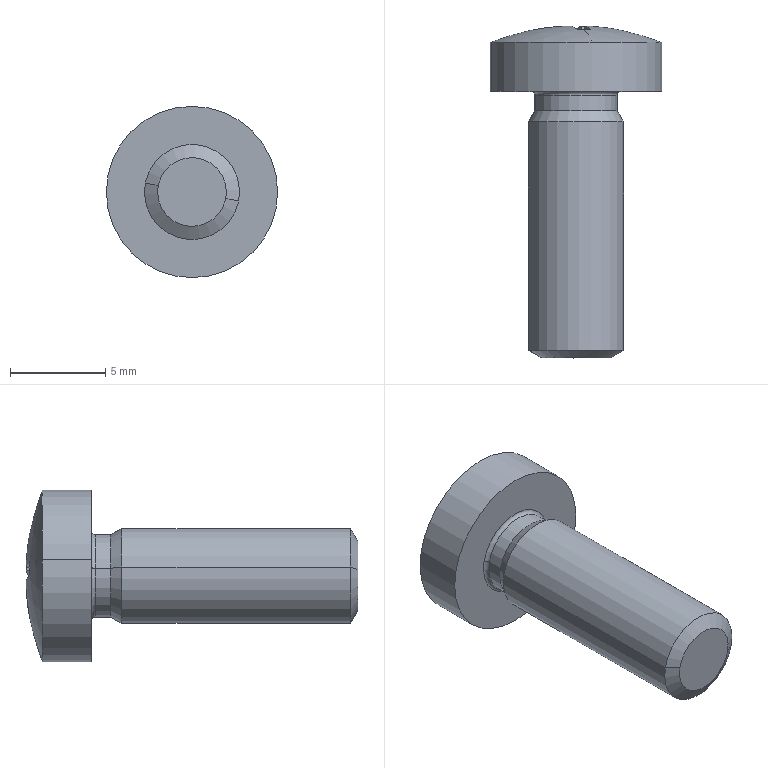Component | SolidWorks | GB823-88PhillipsSmallPanHeadScrewM5_14-1 | 1 solid | 28 faces | box 9 x 17.44 x 9 mm | volume 453 mm3 | plane 14 | cylinder 6 | cone 4 | torus 2 | sphere 2 | commonest cylinder face diameters 4.33 x2 9 x2 5 x2
STEP:
#1=COLOUR_RGB('',0.7922,0.8196,0.9333);
#2=FILL_AREA_STYLE_COLOUR('',#1);
#3=FILL_AREA_STYLE('',(#2));
#4=SURFACE_STYLE_FILL_AREA(#3);
#5=SURFACE_SIDE_STYLE('',(#4));
#6=SURFACE_STYLE_USAGE(.BOTH.,#5);
#7=PRESENTATION_STYLE_ASSIGNMENT((#6));
#8=CARTESIAN_POINT('',(-4.855,2.688,-4.337));
#9=VERTEX_POINT('',#8);
#10=CARTESIAN_POINT('',(-4.715,2.688,-4.364));
#11=VERTEX_POINT('',#10);
#12=CARTESIAN_POINT('',(-4.785,2.688,-4.351));
#13=DIRECTION('',(0.,1.,0.));
#14=DIRECTION('',(-0.9822,0.,0.188));
#15=AXIS2_PLACEMENT_3D('',#12,#13,#14);
#16=CIRCLE('',#15,0.07115);
#17=EDGE_CURVE('',#9,#11,#16,.T.);
#18=ORIENTED_EDGE('',*,*,#17,.T.);
#19=CARTESIAN_POINT('',(-4.688,2.704,-4.369));
#20=VERTEX_POINT('',#19);
#21=CARTESIAN_POINT('',(-4.688,2.704,-4.369));
#22=DIRECTION('',(0.8483,0.5041,-0.1623));
#23=VECTOR('',#22,39.37);
#24=LINE('',#21,#23);
#25=EDGE_CURVE('',#11,#20,#24,.T.);
#26=ORIENTED_EDGE('',*,*,#25,.T.);
#27=CARTESIAN_POINT('',(-4.881,2.704,-4.332));
#28=VERTEX_POINT('',#27);
#29=CARTESIAN_POINT('',(-4.785,2.704,-4.351));
#30=DIRECTION('',(0.,1.,0.));
#31=DIRECTION('',(-0.9822,0.,0.188));
#32=AXIS2_PLACEMENT_3D('',#29,#30,#31);
#33=CIRCLE('',#32,0.09843);
#34=EDGE_CURVE('',#28,#20,#33,.T.);
#35=ORIENTED_EDGE('',*,*,#34,.F.);
#36=CARTESIAN_POINT('',(-4.881,2.704,-4.332));
#37=DIRECTION('',(-0.8483,0.5041,0.1623));
#38=VECTOR('',#37,39.37);
#39=LINE('',#36,#38);
#40=EDGE_CURVE('',#9,#28,#39,.T.);
#41=ORIENTED_EDGE('',*,*,#40,.F.);
#42=EDGE_LOOP('',(#18,#26,#35,#41));
#43=FACE_OUTER_BOUND('',#42,.T.);
#44=CARTESIAN_POINT('',(-4.785,2.704,-4.351));
#45=DIRECTION('',(0.,1.,0.));
#46=DIRECTION('',(-0.9822,0.,0.188));
#47=AXIS2_PLACEMENT_3D('',#44,#45,#46);
#48=CONICAL_SURFACE('',#47,0.09843,1.043);
#49=ADVANCED_FACE('',(#43),#48,.T.);
#50=CARTESIAN_POINT('',(-4.693,3.239,-4.368));
#51=VERTEX_POINT('',#50);
#52=CARTESIAN_POINT('',(-4.876,3.239,-4.333));
#53=VERTEX_POINT('',#52);
#54=CARTESIAN_POINT('',(-4.785,3.239,-4.351));
#55=DIRECTION('',(0.,1.,0.));
#56=DIRECTION('',(-0.9822,0.,0.188));
#57=AXIS2_PLACEMENT_3D('',#54,#55,#56);
#58=CIRCLE('',#57,0.09311);
#59=EDGE_CURVE('',#51,#53,#58,.T.);
#60=ORIENTED_EDGE('',*,*,#59,.F.);
#61=CARTESIAN_POINT('',(-4.701,3.231,-4.367));
#62=VERTEX_POINT('',#61);
#63=CARTESIAN_POINT('',(-4.693,3.231,-4.368));
#64=DIRECTION('',(0.188,0.,0.9822));
#65=DIRECTION('',(0.9822,0.,-0.188));
#66=AXIS2_PLACEMENT_3D('',#63,#64,#65);
#67=CIRCLE('',#66,0.007874);
#68=EDGE_CURVE('',#51,#62,#67,.T.);
#69=ORIENTED_EDGE('',*,*,#68,.T.);
#70=CARTESIAN_POINT('',(-4.869,3.231,-4.335));
#71=VERTEX_POINT('',#70);
#72=CARTESIAN_POINT('',(-4.785,3.231,-4.351));
#73=DIRECTION('',(0.,-1.,0.));
#74=DIRECTION('',(-0.9822,0.,0.188));
#75=AXIS2_PLACEMENT_3D('',#72,#73,#74);
#76=CIRCLE('',#75,0.08524);
#77=EDGE_CURVE('',#71,#62,#76,.T.);
#78=ORIENTED_EDGE('',*,*,#77,.F.);
#79=CARTESIAN_POINT('',(-4.876,3.231,-4.333));
#80=DIRECTION('',(-0.188,0.,-0.9822));
#81=DIRECTION('',(-0.9822,0.,0.188));
#82=AXIS2_PLACEMENT_3D('',#79,#80,#81);
#83=CIRCLE('',#82,0.007874);
#84=EDGE_CURVE('',#53,#71,#83,.T.);
#85=ORIENTED_EDGE('',*,*,#84,.F.);
#86=EDGE_LOOP('',(#60,#69,#78,#85));
#87=FACE_OUTER_BOUND('',#86,.T.);
#88=CARTESIAN_POINT('',(-4.785,3.231,-4.351));
#89=DIRECTION('',(0.,1.,0.));
#90=DIRECTION('',(-0.9822,0.,0.188));
#91=AXIS2_PLACEMENT_3D('',#88,#89,#90);
#92=TOROIDAL_SURFACE('',#91,0.09311,0.007874);
#93=ADVANCED_FACE('',(#87),#92,.F.);
#94=CARTESIAN_POINT('',(-4.869,3.199,-4.335));
#95=VERTEX_POINT('',#94);
#96=CARTESIAN_POINT('',(-4.701,3.199,-4.367));
#97=VERTEX_POINT('',#96);
#98=CARTESIAN_POINT('',(-4.785,3.199,-4.351));
#99=DIRECTION('',(0.,1.,0.));
#100=DIRECTION('',(-0.9822,0.,0.188));
#101=AXIS2_PLACEMENT_3D('',#98,#99,#100);
#102=CIRCLE('',#101,0.08524);
#103=EDGE_CURVE('',#95,#97,#102,.T.);
#104=ORIENTED_EDGE('',*,*,#103,.F.);
#105=CARTESIAN_POINT('',(-4.881,3.176,-4.332));
#106=VERTEX_POINT('',#105);
#107=CARTESIAN_POINT('',(-4.881,3.176,-4.332));
#108=DIRECTION('',(-0.4911,-0.866,0.09398));
#109=VECTOR('',#108,39.37);
#110=LINE('',#107,#109);
#111=EDGE_CURVE('',#95,#106,#110,.T.);
#112=ORIENTED_EDGE('',*,*,#111,.T.);
#113=CARTESIAN_POINT('',(-4.688,3.176,-4.369));
#114=VERTEX_POINT('',#113);
#115=CARTESIAN_POINT('',(-4.785,3.176,-4.351));
#116=DIRECTION('',(0.,1.,0.));
#117=DIRECTION('',(-0.9822,0.,0.188));
#118=AXIS2_PLACEMENT_3D('',#115,#116,#117);
#119=CIRCLE('',#118,0.09843);
#120=EDGE_CURVE('',#106,#114,#119,.T.);
#121=ORIENTED_EDGE('',*,*,#120,.T.);
#122=CARTESIAN_POINT('',(-4.688,3.176,-4.369));
#123=DIRECTION('',(0.4911,-0.866,-0.09398));
#124=VECTOR('',#123,39.37);
#125=LINE('',#122,#124);
#126=EDGE_CURVE('',#97,#114,#125,.T.);
#127=ORIENTED_EDGE('',*,*,#126,.F.);
#128=EDGE_LOOP('',(#104,#112,#121,#127));
#129=FACE_OUTER_BOUND('',#128,.T.);
#130=CARTESIAN_POINT('',(-4.785,3.176,-4.351));
#131=DIRECTION('',(0.,-1.,0.));
#132=DIRECTION('',(0.9822,0.,-0.188));
#133=AXIS2_PLACEMENT_3D('',#130,#131,#132);
#134=CONICAL_SURFACE('',#133,0.09843,0.5236);
#135=ADVANCED_FACE('',(#129),#134,.T.);
#136=ORIENTED_EDGE('',*,*,#103,.T.);
#137=CARTESIAN_POINT('',(-4.701,3.392,-4.367));
#138=DIRECTION('',(0.,1.,0.));
#139=VECTOR('',#138,39.37);
#140=LINE('',#137,#139);
#141=EDGE_CURVE('',#97,#62,#140,.T.);
#142=ORIENTED_EDGE('',*,*,#141,.T.);
#143=CARTESIAN_POINT('',(-4.785,3.231,-4.351));
#144=DIRECTION('',(0.,-1.,0.));
#145=DIRECTION('',(-0.9822,0.,0.188));
#146=AXIS2_PLACEMENT_3D('',#143,#144,#145);
#147=CIRCLE('',#146,0.08524);
#148=EDGE_CURVE('',#62,#71,#147,.T.);
#149=ORIENTED_EDGE('',*,*,#148,.T.);
#150=CARTESIAN_POINT('',(-4.869,3.392,-4.335));
#151=DIRECTION('',(0.,1.,0.));
#152=VECTOR('',#151,39.37);
#153=LINE('',#150,#152);
#154=EDGE_CURVE('',#95,#71,#153,.T.);
#155=ORIENTED_EDGE('',*,*,#154,.F.);
#156=EDGE_LOOP('',(#136,#142,#149,#155));
#157=FACE_OUTER_BOUND('',#156,.T.);
#158=CARTESIAN_POINT('',(-4.785,3.392,-4.351));
#159=DIRECTION('',(0.,1.,0.));
#160=DIRECTION('',(-0.9822,0.,0.188));
#161=AXIS2_PLACEMENT_3D('',#158,#159,#160);
#162=CYLINDRICAL_SURFACE('',#161,0.08524);
#163=ADVANCED_FACE('',(#157),#162,.T.);
#164=CARTESIAN_POINT('',(-4.959,3.239,-4.317));
#165=VERTEX_POINT('',#164);
#166=CARTESIAN_POINT('',(-4.611,3.239,-4.384));
#167=VERTEX_POINT('',#166);
#168=CARTESIAN_POINT('',(-4.785,3.239,-4.351));
#169=DIRECTION('',(0.,1.,0.));
#170=DIRECTION('',(-0.9822,0.,0.188));
#171=AXIS2_PLACEMENT_3D('',#168,#169,#170);
#172=CIRCLE('',#171,0.1772);
#173=EDGE_CURVE('',#165,#167,#172,.T.);
#174=ORIENTED_EDGE('',*,*,#173,.T.);
#175=CARTESIAN_POINT('',(-4.611,3.34,-4.384));
#176=VERTEX_POINT('',#175);
#177=CARTESIAN_POINT('',(-4.611,3.392,-4.384));
#178=DIRECTION('',(0.,1.,0.));
#179=VECTOR('',#178,39.37);
#180=LINE('',#177,#179);
#181=EDGE_CURVE('',#167,#176,#180,.T.);
#182=ORIENTED_EDGE('',*,*,#181,.T.);
#183=CARTESIAN_POINT('',(-4.752,3.34,-4.177));
#184=VERTEX_POINT('',#183);
#185=CARTESIAN_POINT('',(-4.785,3.34,-4.351));
#186=DIRECTION('',(0.,1.,0.));
#187=DIRECTION('',(-0.9822,0.,0.188));
#188=AXIS2_PLACEMENT_3D('',#185,#186,#187);
#189=CIRCLE('',#188,0.1772);
#190=EDGE_CURVE('',#184,#176,#189,.T.);
#191=ORIENTED_EDGE('',*,*,#190,.F.);
#192=CARTESIAN_POINT('',(-4.959,3.34,-4.317));
#193=VERTEX_POINT('',#192);
#194=CARTESIAN_POINT('',(-4.785,3.34,-4.351));
#195=DIRECTION('',(0.,1.,0.));
#196=DIRECTION('',(-0.9822,0.,0.188));
#197=AXIS2_PLACEMENT_3D('',#194,#195,#196);
#198=CIRCLE('',#197,0.1772);
#199=EDGE_CURVE('',#193,#184,#198,.T.);
#200=ORIENTED_EDGE('',*,*,#199,.F.);
#201=CARTESIAN_POINT('',(-4.959,3.392,-4.317));
#202=DIRECTION('',(0.,1.,0.));
#203=VECTOR('',#202,39.37);
#204=LINE('',#201,#203);
#205=EDGE_CURVE('',#165,#193,#204,.T.);
#206=ORIENTED_EDGE('',*,*,#205,.F.);
#207=EDGE_LOOP('',(#174,#182,#191,#200,#206));
#208=FACE_OUTER_BOUND('',#207,.T.);
#209=CARTESIAN_POINT('',(-4.785,3.392,-4.351));
#210=DIRECTION('',(0.,1.,0.));
#211=DIRECTION('',(-0.9822,0.,0.188));
#212=AXIS2_PLACEMENT_3D('',#209,#210,#211);
#213=CYLINDRICAL_SURFACE('',#212,0.1772);
#214=ADVANCED_FACE('',(#208),#213,.T.);
#215=ORIENTED_EDGE('',*,*,#190,.T.);
#216=CARTESIAN_POINT('',(-4.818,3.34,-4.525));
#217=VERTEX_POINT('',#216);
#218=CARTESIAN_POINT('',(-4.785,3.34,-4.351));
#219=DIRECTION('',(0.,1.,0.));
#220=DIRECTION('',(-0.9822,0.,0.188));
#221=AXIS2_PLACEMENT_3D('',#218,#219,#220);
#222=CIRCLE('',#221,0.1772);
#223=EDGE_CURVE('',#176,#217,#222,.T.);
#224=ORIENTED_EDGE('',*,*,#223,.T.);
#225=CARTESIAN_POINT('',(-4.801,3.367,-4.436));
#226=VERTEX_POINT('',#225);
#227=CARTESIAN_POINT('',(-4.785,2.902,-4.351));
#228=DIRECTION('',(0.9822,0.,-0.188));
#229=DIRECTION('',(-0.188,0.,-0.9822));
#230=AXIS2_PLACEMENT_3D('',#227,#228,#229);
#231=CIRCLE('',#230,0.4724);
#232=EDGE_CURVE('',#217,#226,#231,.T.);
#233=ORIENTED_EDGE('',*,*,#232,.T.);
#234=CARTESIAN_POINT('',(-4.787,3.366,-4.439));
#235=VERTEX_POINT('',#234);
#236=CARTESIAN_POINT('',(-4.751,3.061,-4.173));
#237=DIRECTION('',(0.1412,0.6603,0.7377));
#238=DIRECTION('',(-0.1241,0.751,-0.6485));
#239=AXIS2_PLACEMENT_3D('',#236,#237,#238);
#240=CIRCLE('',#239,0.4064);
#241=EDGE_CURVE('',#235,#226,#240,.T.);
#242=ORIENTED_EDGE('',*,*,#241,.F.);
#243=CARTESIAN_POINT('',(-4.772,3.374,-4.369));
#244=VERTEX_POINT('',#243);
#245=CARTESIAN_POINT('',(-4.836,2.91,-4.341));
#246=DIRECTION('',(-0.9718,0.145,0.186));
#247=DIRECTION('',(-0.1424,-0.9894,0.02725));
#248=AXIS2_PLACEMENT_3D('',#245,#246,#247);
#249=CIRCLE('',#248,0.4695);
#250=EDGE_CURVE('',#244,#235,#249,.T.);
#251=ORIENTED_EDGE('',*,*,#250,.F.);
#252=CARTESIAN_POINT('',(-4.702,3.366,-4.381));
#253=VERTEX_POINT('',#252);
#254=CARTESIAN_POINT('',(-4.775,2.91,-4.299));
#255=DIRECTION('',(0.186,0.145,0.9718));
#256=DIRECTION('',(-0.02725,0.9894,-0.1424));
#257=AXIS2_PLACEMENT_3D('',#254,#255,#256);
#258=CIRCLE('',#257,0.4695);
#259=EDGE_CURVE('',#253,#244,#258,.T.);
#260=ORIENTED_EDGE('',*,*,#259,.F.);
#261=CARTESIAN_POINT('',(-4.696,3.366,-4.353));
#262=VERTEX_POINT('',#261);
#263=CARTESIAN_POINT('',(-4.963,3.061,-4.317));
#264=DIRECTION('',(-0.7377,0.6603,0.1412));
#265=DIRECTION('',(-0.6485,-0.751,0.1241));
#266=AXIS2_PLACEMENT_3D('',#263,#264,#265);
#267=CIRCLE('',#266,0.4064);
#268=EDGE_CURVE('',#262,#253,#267,.T.);
#269=ORIENTED_EDGE('',*,*,#268,.F.);
#270=CARTESIAN_POINT('',(-4.766,3.374,-4.338));
#271=VERTEX_POINT('',#270);
#272=CARTESIAN_POINT('',(-4.795,2.91,-4.402));
#273=DIRECTION('',(-0.186,0.145,-0.9718));
#274=DIRECTION('',(-0.02725,-0.9894,-0.1424));
#275=AXIS2_PLACEMENT_3D('',#272,#273,#274);
#276=CIRCLE('',#275,0.4695);
#277=EDGE_CURVE('',#271,#262,#276,.T.);
#278=ORIENTED_EDGE('',*,*,#277,.F.);
#279=CARTESIAN_POINT('',(-4.754,3.366,-4.268));
#280=VERTEX_POINT('',#279);
#281=CARTESIAN_POINT('',(-4.836,2.91,-4.341));
#282=DIRECTION('',(-0.9718,0.145,0.186));
#283=DIRECTION('',(-0.1424,-0.9894,0.02725));
#284=AXIS2_PLACEMENT_3D('',#281,#282,#283);
#285=CIRCLE('',#284,0.4695);
#286=EDGE_CURVE('',#280,#271,#285,.T.);
#287=ORIENTED_EDGE('',*,*,#286,.F.);
#288=CARTESIAN_POINT('',(-4.768,3.367,-4.265));
#289=VERTEX_POINT('',#288);
#290=CARTESIAN_POINT('',(-4.819,3.061,-4.528));
#291=DIRECTION('',(-0.1412,0.6603,-0.7377));
#292=DIRECTION('',(-0.1241,-0.751,-0.6485));
#293=AXIS2_PLACEMENT_3D('',#290,#291,#292);
#294=CIRCLE('',#293,0.4064);
#295=EDGE_CURVE('',#289,#280,#294,.T.);
#296=ORIENTED_EDGE('',*,*,#295,.F.);
#297=CARTESIAN_POINT('',(-4.785,2.902,-4.351));
#298=DIRECTION('',(-0.9822,0.,0.188));
#299=DIRECTION('',(0.188,0.,0.9822));
#300=AXIS2_PLACEMENT_3D('',#297,#298,#299);
#301=CIRCLE('',#300,0.4724);
#302=EDGE_CURVE('',#184,#289,#301,.T.);
#303=ORIENTED_EDGE('',*,*,#302,.F.);
#304=EDGE_LOOP('',(#215,#224,#233,#242,#251,#260,#269,#278,#287,#296,#303));
#305=FACE_OUTER_BOUND('',#304,.T.);
#306=CARTESIAN_POINT('',(-4.785,2.902,-4.351));
#307=DIRECTION('',(0.9822,0.,-0.188));
#308=DIRECTION('',(0.188,0.,0.9822));
#309=AXIS2_PLACEMENT_3D('',#306,#307,#308);
#310=SPHERICAL_SURFACE('',#309,0.4724);
#311=ADVANCED_FACE('',(#305),#310,.T.);
#312=ORIENTED_EDGE('',*,*,#34,.T.);
#313=CARTESIAN_POINT('',(-4.688,3.392,-4.369));
#314=DIRECTION('',(0.,1.,0.));
#315=VECTOR('',#314,39.37);
#316=LINE('',#313,#315);
#317=EDGE_CURVE('',#20,#114,#316,.T.);
#318=ORIENTED_EDGE('',*,*,#317,.T.);
#319=ORIENTED_EDGE('',*,*,#120,.F.);
#320=CARTESIAN_POINT('',(-4.881,3.392,-4.332));
#321=DIRECTION('',(0.,1.,0.));
#322=VECTOR('',#321,39.37);
#323=LINE('',#320,#322);
#324=EDGE_CURVE('',#28,#106,#323,.T.);
#325=ORIENTED_EDGE('',*,*,#324,.F.);
#326=EDGE_LOOP('',(#312,#318,#319,#325));
#327=FACE_OUTER_BOUND('',#326,.T.);
#328=CARTESIAN_POINT('',(-4.785,3.392,-4.351));
#329=DIRECTION('',(0.,1.,0.));
#330=DIRECTION('',(-0.9822,0.,0.188));
#331=AXIS2_PLACEMENT_3D('',#328,#329,#330);
#332=CYLINDRICAL_SURFACE('',#331,0.09843);
#333=ADVANCED_FACE('',(#327),#332,.T.);
#334=ORIENTED_EDGE('',*,*,#317,.F.);
#335=CARTESIAN_POINT('',(-4.785,2.704,-4.351));
#336=DIRECTION('',(0.,1.,0.));
#337=DIRECTION('',(-0.9822,0.,0.188));
#338=AXIS2_PLACEMENT_3D('',#335,#336,#337);
#339=CIRCLE('',#338,0.09843);
#340=EDGE_CURVE('',#20,#28,#339,.T.);
#341=ORIENTED_EDGE('',*,*,#340,.T.);
#342=ORIENTED_EDGE('',*,*,#324,.T.);
#343=CARTESIAN_POINT('',(-4.785,3.176,-4.351));
#344=DIRECTION('',(0.,1.,0.));
#345=DIRECTION('',(-0.9822,0.,0.188));
#346=AXIS2_PLACEMENT_3D('',#343,#344,#345);
#347=CIRCLE('',#346,0.09843);
#348=EDGE_CURVE('',#114,#106,#347,.T.);
#349=ORIENTED_EDGE('',*,*,#348,.F.);
#350=EDGE_LOOP('',(#334,#341,#342,#349));
#351=FACE_OUTER_BOUND('',#350,.T.);
#352=CARTESIAN_POINT('',(-4.785,3.392,-4.351));
#353=DIRECTION('',(0.,1.,0.));
#354=DIRECTION('',(-0.9822,0.,0.188));
#355=AXIS2_PLACEMENT_3D('',#352,#353,#354);
#356=CYLINDRICAL_SURFACE('',#355,0.09843);
#357=ADVANCED_FACE('',(#351),#356,.T.);
#358=ORIENTED_EDGE('',*,*,#232,.F.);
#359=CARTESIAN_POINT('',(-4.785,3.34,-4.351));
#360=DIRECTION('',(0.,1.,0.));
#361=DIRECTION('',(-0.9822,0.,0.188));
#362=AXIS2_PLACEMENT_3D('',#359,#360,#361);
#363=CIRCLE('',#362,0.1772);
#364=EDGE_CURVE('',#217,#193,#363,.T.);
#365=ORIENTED_EDGE('',*,*,#364,.T.);
#366=ORIENTED_EDGE('',*,*,#199,.T.);
#367=ORIENTED_EDGE('',*,*,#302,.T.);
#368=CARTESIAN_POINT('',(-4.783,3.366,-4.262));
#369=VERTEX_POINT('',#368);
#370=CARTESIAN_POINT('',(-4.819,3.061,-4.528));
#371=DIRECTION('',(-0.1412,0.6603,-0.7377));
#372=DIRECTION('',(-0.1241,-0.751,-0.6485));
#373=AXIS2_PLACEMENT_3D('',#370,#371,#372);
#374=CIRCLE('',#373,0.4064);
#375=EDGE_CURVE('',#369,#289,#374,.T.);
#376=ORIENTED_EDGE('',*,*,#375,.F.);
#377=CARTESIAN_POINT('',(-4.797,3.374,-4.332));
#378=VERTEX_POINT('',#377);
#379=CARTESIAN_POINT('',(-4.733,2.91,-4.361));
#380=DIRECTION('',(0.9718,0.145,-0.186));
#381=DIRECTION('',(-0.1424,0.9894,0.02725));
#382=AXIS2_PLACEMENT_3D('',#379,#380,#381);
#383=CIRCLE('',#382,0.4695);
#384=EDGE_CURVE('',#378,#369,#383,.T.);
#385=ORIENTED_EDGE('',*,*,#384,.F.);
#386=CARTESIAN_POINT('',(-4.868,3.366,-4.32));
#387=VERTEX_POINT('',#386);
#388=CARTESIAN_POINT('',(-4.795,2.91,-4.402));
#389=DIRECTION('',(-0.186,0.145,-0.9718));
#390=DIRECTION('',(-0.02725,-0.9894,-0.1424));
#391=AXIS2_PLACEMENT_3D('',#388,#389,#390);
#392=CIRCLE('',#391,0.4695);
#393=EDGE_CURVE('',#387,#378,#392,.T.);
#394=ORIENTED_EDGE('',*,*,#393,.F.);
#395=CARTESIAN_POINT('',(-4.873,3.366,-4.349));
#396=VERTEX_POINT('',#395);
#397=CARTESIAN_POINT('',(-4.607,3.061,-4.385));
#398=DIRECTION('',(0.7377,0.6603,-0.1412));
#399=DIRECTION('',(-0.6485,0.751,0.1241));
#400=AXIS2_PLACEMENT_3D('',#397,#398,#399);
#401=CIRCLE('',#400,0.4064);
#402=EDGE_CURVE('',#396,#387,#401,.T.);
#403=ORIENTED_EDGE('',*,*,#402,.F.);
#404=CARTESIAN_POINT('',(-4.803,3.374,-4.363));
#405=VERTEX_POINT('',#404);
#406=CARTESIAN_POINT('',(-4.775,2.91,-4.299));
#407=DIRECTION('',(0.186,0.145,0.9718));
#408=DIRECTION('',(-0.02725,0.9894,-0.1424));
#409=AXIS2_PLACEMENT_3D('',#406,#407,#408);
#410=CIRCLE('',#409,0.4695);
#411=EDGE_CURVE('',#405,#396,#410,.T.);
#412=ORIENTED_EDGE('',*,*,#411,.F.);
#413=CARTESIAN_POINT('',(-4.815,3.366,-4.434));
#414=VERTEX_POINT('',#413);
#415=CARTESIAN_POINT('',(-4.733,2.91,-4.361));
#416=DIRECTION('',(0.9718,0.145,-0.186));
#417=DIRECTION('',(-0.1424,0.9894,0.02725));
#418=AXIS2_PLACEMENT_3D('',#415,#416,#417);
#419=CIRCLE('',#418,0.4695);
#420=EDGE_CURVE('',#414,#405,#419,.T.);
#421=ORIENTED_EDGE('',*,*,#420,.F.);
#422=CARTESIAN_POINT('',(-4.751,3.061,-4.173));
#423=DIRECTION('',(0.1412,0.6603,0.7377));
#424=DIRECTION('',(-0.1241,0.751,-0.6485));
#425=AXIS2_PLACEMENT_3D('',#422,#423,#424);
#426=CIRCLE('',#425,0.4064);
#427=EDGE_CURVE('',#226,#414,#426,.T.);
#428=ORIENTED_EDGE('',*,*,#427,.F.);
#429=EDGE_LOOP('',(#358,#365,#366,#367,#376,#385,#394,#403,#412,#421,#428));
#430=FACE_OUTER_BOUND('',#429,.T.);
#431=CARTESIAN_POINT('',(-4.785,2.902,-4.351));
#432=DIRECTION('',(0.9822,0.,-0.188));
#433=DIRECTION('',(0.188,0.,0.9822));
#434=AXIS2_PLACEMENT_3D('',#431,#432,#433);
#435=SPHERICAL_SURFACE('',#434,0.4724);
#436=ADVANCED_FACE('',(#430),#435,.T.);
#437=ORIENTED_EDGE('',*,*,#286,.T.);
#438=CARTESIAN_POINT('',(-4.785,3.267,-4.351));
#439=VERTEX_POINT('',#438);
#440=CARTESIAN_POINT('',(-4.785,3.267,-4.351));
#441=DIRECTION('',(-0.1679,-0.9792,-0.1139));
#442=VECTOR('',#441,39.37);
#443=LINE('',#440,#442);
#444=EDGE_CURVE('',#271,#439,#443,.T.);
#445=ORIENTED_EDGE('',*,*,#444,.T.);
#446=CARTESIAN_POINT('',(-4.752,3.375,-4.261));
#447=DIRECTION('',(-0.2308,-0.7465,-0.624));
#448=VECTOR('',#447,39.37);
#449=LINE('',#446,#448);
#450=EDGE_CURVE('',#280,#439,#449,.T.);
#451=ORIENTED_EDGE('',*,*,#450,.F.);
#452=EDGE_LOOP('',(#437,#445,#451));
#453=FACE_OUTER_BOUND('',#452,.T.);
#454=CARTESIAN_POINT('',(-4.785,3.267,-4.351));
#455=DIRECTION('',(-0.9718,0.145,0.186));
#456=DIRECTION('',(-0.1424,-0.9894,0.02725));
#457=AXIS2_PLACEMENT_3D('',#454,#455,#456);
#458=PLANE('',#457);
#459=ADVANCED_FACE('',(#453),#458,.T.);
#460=CARTESIAN_POINT('',(-4.787,3.375,-4.446));
#461=DIRECTION('',(0.01593,-0.7465,0.6652));
#462=VECTOR('',#461,39.37);
#463=LINE('',#460,#462);
#464=EDGE_CURVE('',#235,#439,#463,.T.);
#465=ORIENTED_EDGE('',*,*,#464,.T.);
#466=CARTESIAN_POINT('',(-4.785,3.267,-4.351));
#467=DIRECTION('',(0.1139,0.9792,-0.1679));
#468=VECTOR('',#467,39.37);
#469=LINE('',#466,#468);
#470=EDGE_CURVE('',#439,#244,#469,.T.);
#471=ORIENTED_EDGE('',*,*,#470,.T.);
#472=ORIENTED_EDGE('',*,*,#250,.T.);
#473=EDGE_LOOP('',(#465,#471,#472));
#474=FACE_OUTER_BOUND('',#473,.T.);
#475=CARTESIAN_POINT('',(-4.785,3.267,-4.351));
#476=DIRECTION('',(-0.9718,0.145,0.186));
#477=DIRECTION('',(-0.1424,-0.9894,0.02725));
#478=AXIS2_PLACEMENT_3D('',#475,#476,#477);
#479=PLANE('',#478);
#480=ADVANCED_FACE('',(#474),#479,.T.);
#481=CARTESIAN_POINT('',(-4.783,3.375,-4.255));
#482=DIRECTION('',(-0.01593,-0.7465,-0.6652));
#483=VECTOR('',#482,39.37);
#484=LINE('',#481,#483);
#485=EDGE_CURVE('',#369,#439,#484,.T.);
#486=ORIENTED_EDGE('',*,*,#485,.T.);
#487=CARTESIAN_POINT('',(-4.785,3.267,-4.351));
#488=DIRECTION('',(-0.1139,0.9792,0.1679));
#489=VECTOR('',#488,39.37);
#490=LINE('',#487,#489);
#491=EDGE_CURVE('',#439,#378,#490,.T.);
#492=ORIENTED_EDGE('',*,*,#491,.T.);
#493=ORIENTED_EDGE('',*,*,#384,.T.);
#494=EDGE_LOOP('',(#486,#492,#493));
#495=FACE_OUTER_BOUND('',#494,.T.);
#496=CARTESIAN_POINT('',(-4.785,3.267,-4.351));
#497=DIRECTION('',(0.9718,0.145,-0.186));
#498=DIRECTION('',(-0.1424,0.9894,0.02725));
#499=AXIS2_PLACEMENT_3D('',#496,#497,#498);
#500=PLANE('',#499);
#501=ADVANCED_FACE('',(#495),#500,.T.);
#502=ORIENTED_EDGE('',*,*,#420,.T.);
#503=CARTESIAN_POINT('',(-4.785,3.267,-4.351));
#504=DIRECTION('',(0.1679,-0.9792,0.1139));
#505=VECTOR('',#504,39.37);
#506=LINE('',#503,#505);
#507=EDGE_CURVE('',#405,#439,#506,.T.);
#508=ORIENTED_EDGE('',*,*,#507,.T.);
#509=CARTESIAN_POINT('',(-4.818,3.375,-4.441));
#510=DIRECTION('',(0.2308,-0.7465,0.624));
#511=VECTOR('',#510,39.37);
#512=LINE('',#509,#511);
#513=EDGE_CURVE('',#414,#439,#512,.T.);
#514=ORIENTED_EDGE('',*,*,#513,.F.);
#515=EDGE_LOOP('',(#502,#508,#514));
#516=FACE_OUTER_BOUND('',#515,.T.);
#517=CARTESIAN_POINT('',(-4.785,3.267,-4.351));
#518=DIRECTION('',(0.9718,0.145,-0.186));
#519=DIRECTION('',(-0.1424,0.9894,0.02725));
#520=AXIS2_PLACEMENT_3D('',#517,#518,#519);
#521=PLANE('',#520);
#522=ADVANCED_FACE('',(#516),#521,.T.);
#523=ORIENTED_EDGE('',*,*,#181,.F.);
#524=CARTESIAN_POINT('',(-4.785,3.239,-4.351));
#525=DIRECTION('',(0.,1.,0.));
#526=DIRECTION('',(-0.9822,0.,0.188));
#527=AXIS2_PLACEMENT_3D('',#524,#525,#526);
#528=CIRCLE('',#527,0.1772);
#529=EDGE_CURVE('',#167,#165,#528,.T.);
#530=ORIENTED_EDGE('',*,*,#529,.T.);
#531=ORIENTED_EDGE('',*,*,#205,.T.);
#532=ORIENTED_EDGE('',*,*,#364,.F.);
#533=ORIENTED_EDGE('',*,*,#223,.F.);
#534=EDGE_LOOP('',(#523,#530,#531,#532,#533));
#535=FACE_OUTER_BOUND('',#534,.T.);
#536=CARTESIAN_POINT('',(-4.785,3.392,-4.351));
#537=DIRECTION('',(0.,1.,0.));
#538=DIRECTION('',(-0.9822,0.,0.188));
#539=AXIS2_PLACEMENT_3D('',#536,#537,#538);
#540=CYLINDRICAL_SURFACE('',#539,0.1772);
#541=ADVANCED_FACE('',(#535),#540,.T.);
#542=CARTESIAN_POINT('',(-4.785,3.239,-4.351));
#543=DIRECTION('',(0.,1.,0.));
#544=DIRECTION('',(-0.9822,0.,0.188));
#545=AXIS2_PLACEMENT_3D('',#542,#543,#544);
#546=CIRCLE('',#545,0.09311);
#547=EDGE_CURVE('',#53,#51,#546,.T.);
#548=ORIENTED_EDGE('',*,*,#547,.T.);
#549=ORIENTED_EDGE('',*,*,#59,.T.);
#550=EDGE_LOOP('',(#548,#549));
#551=FACE_BOUND('',#550,.T.);
#552=ORIENTED_EDGE('',*,*,#173,.F.);
#553=ORIENTED_EDGE('',*,*,#529,.F.);
#554=EDGE_LOOP('',(#552,#553));
#555=FACE_OUTER_BOUND('',#554,.T.);
#556=CARTESIAN_POINT('',(-4.769,3.239,-4.267));
#557=DIRECTION('',(0.,1.,0.));
#558=DIRECTION('',(-0.9822,0.,0.188));
#559=AXIS2_PLACEMENT_3D('',#556,#557,#558);
#560=PLANE('',#559);
#561=ADVANCED_FACE('',(#551,#555),#560,.F.);
#562=ORIENTED_EDGE('',*,*,#141,.F.);
#563=CARTESIAN_POINT('',(-4.785,3.199,-4.351));
#564=DIRECTION('',(0.,1.,0.));
#565=DIRECTION('',(-0.9822,0.,0.188));
#566=AXIS2_PLACEMENT_3D('',#563,#564,#565);
#567=CIRCLE('',#566,0.08524);
#568=EDGE_CURVE('',#97,#95,#567,.T.);
#569=ORIENTED_EDGE('',*,*,#568,.T.);
#570=ORIENTED_EDGE('',*,*,#154,.T.);
#571=ORIENTED_EDGE('',*,*,#77,.T.);
#572=EDGE_LOOP('',(#562,#569,#570,#571));
#573=FACE_OUTER_BOUND('',#572,.T.);
#574=CARTESIAN_POINT('',(-4.785,3.392,-4.351));
#575=DIRECTION('',(0.,1.,0.));
#576=DIRECTION('',(-0.9822,0.,0.188));
#577=AXIS2_PLACEMENT_3D('',#574,#575,#576);
#578=CYLINDRICAL_SURFACE('',#577,0.08524);
#579=ADVANCED_FACE('',(#573),#578,.T.);
#580=ORIENTED_EDGE('',*,*,#111,.F.);
#581=ORIENTED_EDGE('',*,*,#568,.F.);
#582=ORIENTED_EDGE('',*,*,#126,.T.);
#583=ORIENTED_EDGE('',*,*,#348,.T.);
#584=EDGE_LOOP('',(#580,#581,#582,#583));
#585=FACE_OUTER_BOUND('',#584,.T.);
#586=CARTESIAN_POINT('',(-4.785,3.176,-4.351));
#587=DIRECTION('',(0.,-1.,0.));
#588=DIRECTION('',(0.9822,0.,-0.188));
#589=AXIS2_PLACEMENT_3D('',#586,#587,#588);
#590=CONICAL_SURFACE('',#589,0.09843,0.5236);
#591=ADVANCED_FACE('',(#585),#590,.T.);
#592=ORIENTED_EDGE('',*,*,#68,.F.);
#593=ORIENTED_EDGE('',*,*,#547,.F.);
#594=ORIENTED_EDGE('',*,*,#84,.T.);
#595=ORIENTED_EDGE('',*,*,#148,.F.);
#596=EDGE_LOOP('',(#592,#593,#594,#595));
#597=FACE_OUTER_BOUND('',#596,.T.);
#598=CARTESIAN_POINT('',(-4.785,3.231,-4.351));
#599=DIRECTION('',(0.,1.,0.));
#600=DIRECTION('',(-0.9822,0.,0.188));
#601=AXIS2_PLACEMENT_3D('',#598,#599,#600);
#602=TOROIDAL_SURFACE('',#601,0.09311,0.007874);
#603=ADVANCED_FACE('',(#597),#602,.F.);
#604=ORIENTED_EDGE('',*,*,#375,.T.);
#605=ORIENTED_EDGE('',*,*,#295,.T.);
#606=ORIENTED_EDGE('',*,*,#450,.T.);
#607=ORIENTED_EDGE('',*,*,#485,.F.);
#608=EDGE_LOOP('',(#604,#605,#606,#607));
#609=FACE_OUTER_BOUND('',#608,.T.);
#610=CARTESIAN_POINT('',(-4.783,3.375,-4.255));
#611=DIRECTION('',(-0.1412,0.6603,-0.7377));
#612=DIRECTION('',(-0.1241,-0.751,-0.6485));
#613=AXIS2_PLACEMENT_3D('',#610,#611,#612);
#614=PLANE('',#613);
#615=ADVANCED_FACE('',(#609),#614,.T.);
#616=ORIENTED_EDGE('',*,*,#241,.T.);
#617=ORIENTED_EDGE('',*,*,#427,.T.);
#618=ORIENTED_EDGE('',*,*,#513,.T.);
#619=ORIENTED_EDGE('',*,*,#464,.F.);
#620=EDGE_LOOP('',(#616,#617,#618,#619));
#621=FACE_OUTER_BOUND('',#620,.T.);
#622=CARTESIAN_POINT('',(-4.787,3.375,-4.446));
#623=DIRECTION('',(0.1412,0.6603,0.7377));
#624=DIRECTION('',(-0.1241,0.751,-0.6485));
#625=AXIS2_PLACEMENT_3D('',#622,#623,#624);
#626=PLANE('',#625);
#627=ADVANCED_FACE('',(#621),#626,.T.);
#628=ORIENTED_EDGE('',*,*,#393,.T.);
#629=ORIENTED_EDGE('',*,*,#491,.F.);
#630=CARTESIAN_POINT('',(-4.875,3.375,-4.317));
#631=DIRECTION('',(0.624,-0.7465,-0.2308));
#632=VECTOR('',#631,39.37);
#633=LINE('',#630,#632);
#634=EDGE_CURVE('',#387,#439,#633,.T.);
#635=ORIENTED_EDGE('',*,*,#634,.F.);
#636=EDGE_LOOP('',(#628,#629,#635));
#637=FACE_OUTER_BOUND('',#636,.T.);
#638=CARTESIAN_POINT('',(-4.785,3.267,-4.351));
#639=DIRECTION('',(-0.186,0.145,-0.9718));
#640=DIRECTION('',(-0.02725,-0.9894,-0.1424));
#641=AXIS2_PLACEMENT_3D('',#638,#639,#640);
#642=PLANE('',#641);
#643=ADVANCED_FACE('',(#637),#642,.T.);
#644=ORIENTED_EDGE('',*,*,#411,.T.);
#645=CARTESIAN_POINT('',(-4.881,3.375,-4.348));
#646=DIRECTION('',(0.6652,-0.7465,-0.01593));
#647=VECTOR('',#646,39.37);
#648=LINE('',#645,#647);
#649=EDGE_CURVE('',#396,#439,#648,.T.);
#650=ORIENTED_EDGE('',*,*,#649,.T.);
#651=ORIENTED_EDGE('',*,*,#507,.F.);
#652=EDGE_LOOP('',(#644,#650,#651));
#653=FACE_OUTER_BOUND('',#652,.T.);
#654=CARTESIAN_POINT('',(-4.785,3.267,-4.351));
#655=DIRECTION('',(0.186,0.145,0.9718));
#656=DIRECTION('',(-0.02725,0.9894,-0.1424));
#657=AXIS2_PLACEMENT_3D('',#654,#655,#656);
#658=PLANE('',#657);
#659=ADVANCED_FACE('',(#653),#658,.T.);
#660=ORIENTED_EDGE('',*,*,#402,.T.);
#661=ORIENTED_EDGE('',*,*,#634,.T.);
#662=ORIENTED_EDGE('',*,*,#649,.F.);
#663=EDGE_LOOP('',(#660,#661,#662));
#664=FACE_OUTER_BOUND('',#663,.T.);
#665=CARTESIAN_POINT('',(-4.881,3.375,-4.348));
#666=DIRECTION('',(0.7377,0.6603,-0.1412));
#667=DIRECTION('',(0.6485,-0.751,-0.1241));
#668=AXIS2_PLACEMENT_3D('',#665,#666,#667);
#669=PLANE('',#668);
#670=ADVANCED_FACE('',(#664),#669,.T.);
#671=ORIENTED_EDGE('',*,*,#277,.T.);
#672=CARTESIAN_POINT('',(-4.689,3.375,-4.353));
#673=DIRECTION('',(-0.6652,-0.7465,0.01593));
#674=VECTOR('',#673,39.37);
#675=LINE('',#672,#674);
#676=EDGE_CURVE('',#262,#439,#675,.T.);
#677=ORIENTED_EDGE('',*,*,#676,.T.);
#678=ORIENTED_EDGE('',*,*,#444,.F.);
#679=EDGE_LOOP('',(#671,#677,#678));
#680=FACE_OUTER_BOUND('',#679,.T.);
#681=CARTESIAN_POINT('',(-4.785,3.267,-4.351));
#682=DIRECTION('',(-0.186,0.145,-0.9718));
#683=DIRECTION('',(-0.02725,-0.9894,-0.1424));
#684=AXIS2_PLACEMENT_3D('',#681,#682,#683);
#685=PLANE('',#684);
#686=ADVANCED_FACE('',(#680),#685,.T.);
#687=ORIENTED_EDGE('',*,*,#259,.T.);
#688=ORIENTED_EDGE('',*,*,#470,.F.);
#689=CARTESIAN_POINT('',(-4.695,3.375,-4.384));
#690=DIRECTION('',(-0.624,-0.7465,0.2308));
#691=VECTOR('',#690,39.37);
#692=LINE('',#689,#691);
#693=EDGE_CURVE('',#253,#439,#692,.T.);
#694=ORIENTED_EDGE('',*,*,#693,.F.);
#695=EDGE_LOOP('',(#687,#688,#694));
#696=FACE_OUTER_BOUND('',#695,.T.);
#697=CARTESIAN_POINT('',(-4.785,3.267,-4.351));
#698=DIRECTION('',(0.186,0.145,0.9718));
#699=DIRECTION('',(-0.02725,0.9894,-0.1424));
#700=AXIS2_PLACEMENT_3D('',#697,#698,#699);
#701=PLANE('',#700);
#702=ADVANCED_FACE('',(#696),#701,.T.);
#703=ORIENTED_EDGE('',*,*,#268,.T.);
#704=ORIENTED_EDGE('',*,*,#693,.T.);
#705=ORIENTED_EDGE('',*,*,#676,.F.);
#706=EDGE_LOOP('',(#703,#704,#705));
#707=FACE_OUTER_BOUND('',#706,.T.);
#708=CARTESIAN_POINT('',(-4.689,3.375,-4.353));
#709=DIRECTION('',(-0.7377,0.6603,0.1412));
#710=DIRECTION('',(0.6485,0.751,-0.1241));
#711=AXIS2_PLACEMENT_3D('',#708,#709,#710);
#712=PLANE('',#711);
#713=ADVANCED_FACE('',(#707),#712,.T.);
#714=ORIENTED_EDGE('',*,*,#25,.F.);
#715=CARTESIAN_POINT('',(-4.785,2.688,-4.351));
#716=DIRECTION('',(0.,1.,0.));
#717=DIRECTION('',(-0.9822,0.,0.188));
#718=AXIS2_PLACEMENT_3D('',#715,#716,#717);
#719=CIRCLE('',#718,0.07115);
#720=EDGE_CURVE('',#11,#9,#719,.T.);
#721=ORIENTED_EDGE('',*,*,#720,.T.);
#722=ORIENTED_EDGE('',*,*,#40,.T.);
#723=ORIENTED_EDGE('',*,*,#340,.F.);
#724=EDGE_LOOP('',(#714,#721,#722,#723));
#725=FACE_OUTER_BOUND('',#724,.T.);
#726=CARTESIAN_POINT('',(-4.785,2.704,-4.351));
#727=DIRECTION('',(0.,1.,0.));
#728=DIRECTION('',(-0.9822,0.,0.188));
#729=AXIS2_PLACEMENT_3D('',#726,#727,#728);
#730=CONICAL_SURFACE('',#729,0.09843,1.043);
#731=ADVANCED_FACE('',(#725),#730,.T.);
#732=ORIENTED_EDGE('',*,*,#17,.F.);
#733=ORIENTED_EDGE('',*,*,#720,.F.);
#734=EDGE_LOOP('',(#732,#733));
#735=FACE_OUTER_BOUND('',#734,.T.);
#736=CARTESIAN_POINT('',(-4.785,2.688,-4.351));
#737=DIRECTION('',(0.,1.,0.));
#738=DIRECTION('',(-0.9822,0.,0.188));
#739=AXIS2_PLACEMENT_3D('',#736,#737,#738);
#740=PLANE('',#739);
#741=ADVANCED_FACE('',(#735),#740,.F.);
#742=CLOSED_SHELL('',(#49,#93,#135,#163,#214,#311,#333,#357,#436,#459,#480,#501,#522,#541,#561,#579,#591,#603,#615,#627,#643,#659,#670,#686,#702,#713,#731,#741));
#743=MANIFOLD_SOLID_BREP('',#742);
#744=STYLED_ITEM('',(#7),#743);
#745=PRESENTATION_LAYER_ASSIGNMENT('','',(#744));
#746=(LENGTH_UNIT()NAMED_UNIT(*)SI_UNIT($,.METRE.));
#747=LENGTH_MEASURE_WITH_UNIT(LENGTH_MEASURE(0.0254),#746);
#748=DIMENSIONAL_EXPONENTS(1.,0.,0.,0.,0.,0.,0.);
#749=(CONVERSION_BASED_UNIT('',#747)LENGTH_UNIT()NAMED_UNIT(#748));
#750=UNCERTAINTY_MEASURE_WITH_UNIT(LENGTH_MEASURE(0.00001),#749,'','');
#751=(NAMED_UNIT(*)PLANE_ANGLE_UNIT()SI_UNIT($,.RADIAN.));
#752=(NAMED_UNIT(*)SI_UNIT($,.STERADIAN.)SOLID_ANGLE_UNIT());
#753=(GEOMETRIC_REPRESENTATION_CONTEXT(3)GLOBAL_UNCERTAINTY_ASSIGNED_CONTEXT((#750))GLOBAL_UNIT_ASSIGNED_CONTEXT((#749,#751,#752))REPRESENTATION_CONTEXT('',''));
#754=MECHANICAL_DESIGN_GEOMETRIC_PRESENTATION_REPRESENTATION('',(#744),#753);
#755=CARTESIAN_POINT('',(0.,0.,0.));
#756=DIRECTION('',(0.,0.,1.));
#757=DIRECTION('',(1.,0.,0.));
#758=AXIS2_PLACEMENT_3D('',#755,#756,#757);
#759=(LENGTH_UNIT()NAMED_UNIT(*)SI_UNIT($,.METRE.));
#760=LENGTH_MEASURE_WITH_UNIT(LENGTH_MEASURE(0.0254),#759);
#761=DIMENSIONAL_EXPONENTS(1.,0.,0.,0.,0.,0.,0.);
#762=(CONVERSION_BASED_UNIT('',#760)LENGTH_UNIT()NAMED_UNIT(#761));
#763=UNCERTAINTY_MEASURE_WITH_UNIT(LENGTH_MEASURE(0.00001),#762,'','');
#764=(NAMED_UNIT(*)PLANE_ANGLE_UNIT()SI_UNIT($,.RADIAN.));
#765=(NAMED_UNIT(*)SI_UNIT($,.STERADIAN.)SOLID_ANGLE_UNIT());
#766=(GEOMETRIC_REPRESENTATION_CONTEXT(3)GLOBAL_UNCERTAINTY_ASSIGNED_CONTEXT((#763))GLOBAL_UNIT_ASSIGNED_CONTEXT((#762,#764,#765))REPRESENTATION_CONTEXT('',''));
#767=ADVANCED_BREP_SHAPE_REPRESENTATION('',(#743,#758),#766);